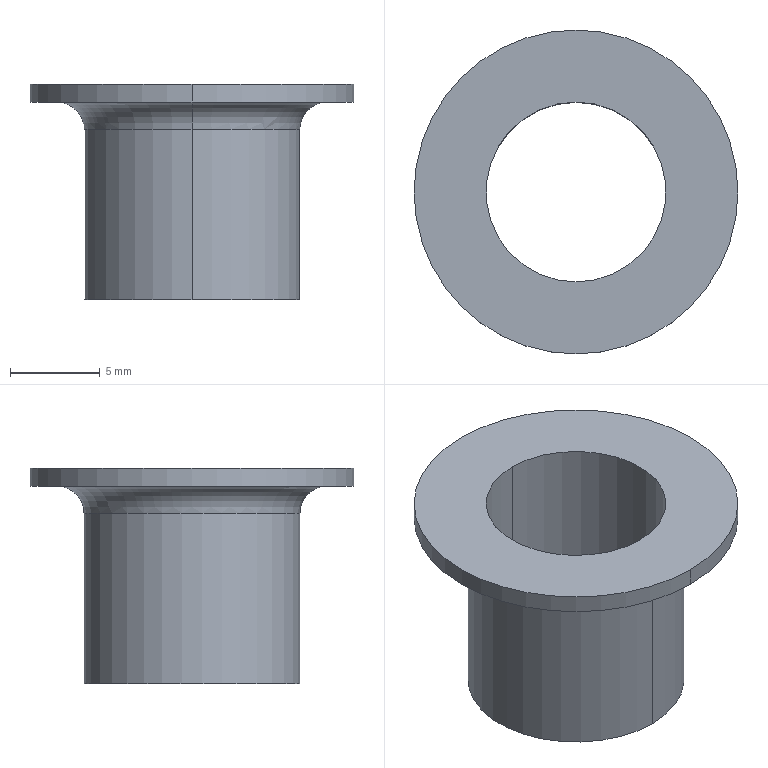Component | SolidWorks | C-SFF10120-1 | 1 solid | 11 faces | box 18 x 18 x 12 mm | volume 575 mm3 | cylinder 6 | plane 3 | torus 2 | commonest cylinder face diameters 12 x2 18 x2 10 x2 | material Tin Bronze
build123d program:
from build123d import *

# Parameters (mm, degrees)
FILLET1_R = 1.5


with BuildPart() as part:
    # Sketch1 → Revolve1 (revolve)
    with BuildSketch(Plane(origin=(0, 0, 0), x_dir=(0, 0, -1), z_dir=(1, 0, 0)), mode=Mode.PRIVATE) as revolve1_sk:
        Polygon((-5, 0), (-9, 0), (-9, 1), (-6, 1), (-6, 12), (-5, 12), align=None)
    revolve(revolve1_sk.sketch.rotate(Axis((0, 0, 0), (0, 1, 0)), 180), axis=Axis((0, 0, 0), (0, 1, 0)))

    # Fillet1
    fillet1_edges = [part.edges().sort_by_distance(p)[0] for p in [
        (0, 1, 6),
    ]]
    fillet(fillet1_edges, radius=FILLET1_R)


solid = part.part

# Placed as in the assembly
solid = solid.moved(Location((31.561, -84.186, 318), (-90, 0, 0)))
STEP:
#1=CARTESIAN_POINT('',(1.243,-3.019,12.48));
#2=VERTEX_POINT('',#1);
#3=CARTESIAN_POINT('',(1.243,-3.61,12.48));
#4=VERTEX_POINT('',#3);
#5=CARTESIAN_POINT('',(1.243,-3.314,12.48));
#6=DIRECTION('',(0.,0.,1.));
#7=DIRECTION('',(0.,-1.,0.));
#8=AXIS2_PLACEMENT_3D('',#5,#6,#7);
#9=CIRCLE('',#8,0.2953);
#10=EDGE_CURVE('',#2,#4,#9,.T.);
#11=ORIENTED_EDGE('',*,*,#10,.F.);
#12=CARTESIAN_POINT('',(1.243,-3.078,12.421));
#13=VERTEX_POINT('',#12);
#14=CARTESIAN_POINT('',(1.243,-3.019,12.421));
#15=DIRECTION('',(1.,-0.,0.));
#16=DIRECTION('',(0.,1.,0.));
#17=AXIS2_PLACEMENT_3D('',#14,#15,#16);
#18=CIRCLE('',#17,0.05906);
#19=EDGE_CURVE('',#2,#13,#18,.T.);
#20=ORIENTED_EDGE('',*,*,#19,.T.);
#21=CARTESIAN_POINT('',(1.243,-3.551,12.421));
#22=VERTEX_POINT('',#21);
#23=CARTESIAN_POINT('',(1.243,-3.314,12.421));
#24=DIRECTION('',(0.,0.,-1.));
#25=DIRECTION('',(0.,-1.,0.));
#26=AXIS2_PLACEMENT_3D('',#23,#24,#25);
#27=CIRCLE('',#26,0.2362);
#28=EDGE_CURVE('',#22,#13,#27,.T.);
#29=ORIENTED_EDGE('',*,*,#28,.F.);
#30=CARTESIAN_POINT('',(1.243,-3.61,12.421));
#31=DIRECTION('',(-1.,0.,0.));
#32=DIRECTION('',(0.,0.,1.));
#33=AXIS2_PLACEMENT_3D('',#30,#31,#32);
#34=CIRCLE('',#33,0.05906);
#35=EDGE_CURVE('',#4,#22,#34,.T.);
#36=ORIENTED_EDGE('',*,*,#35,.F.);
#37=EDGE_LOOP('',(#11,#20,#29,#36));
#38=FACE_OUTER_BOUND('',#37,.T.);
#39=CARTESIAN_POINT('',(1.243,-3.314,12.421));
#40=DIRECTION('',(0.,0.,1.));
#41=DIRECTION('',(0.,-1.,0.));
#42=AXIS2_PLACEMENT_3D('',#39,#40,#41);
#43=TOROIDAL_SURFACE('',#42,0.2953,0.05906);
#44=ADVANCED_FACE('',(#38),#43,.F.);
#45=CARTESIAN_POINT('',(1.243,-3.551,12.047));
#46=VERTEX_POINT('',#45);
#47=CARTESIAN_POINT('',(1.243,-3.078,12.047));
#48=VERTEX_POINT('',#47);
#49=CARTESIAN_POINT('',(1.243,-3.314,12.047));
#50=DIRECTION('',(0.,0.,1.));
#51=DIRECTION('',(0.,-1.,0.));
#52=AXIS2_PLACEMENT_3D('',#49,#50,#51);
#53=CIRCLE('',#52,0.2362);
#54=EDGE_CURVE('',#46,#48,#53,.T.);
#55=ORIENTED_EDGE('',*,*,#54,.T.);
#56=CARTESIAN_POINT('',(1.243,-3.078,12.52));
#57=DIRECTION('',(0.,0.,1.));
#58=VECTOR('',#57,39.37);
#59=LINE('',#56,#58);
#60=EDGE_CURVE('',#48,#13,#59,.T.);
#61=ORIENTED_EDGE('',*,*,#60,.T.);
#62=CARTESIAN_POINT('',(1.243,-3.314,12.421));
#63=DIRECTION('',(0.,0.,-1.));
#64=DIRECTION('',(0.,-1.,0.));
#65=AXIS2_PLACEMENT_3D('',#62,#63,#64);
#66=CIRCLE('',#65,0.2362);
#67=EDGE_CURVE('',#13,#22,#66,.T.);
#68=ORIENTED_EDGE('',*,*,#67,.T.);
#69=CARTESIAN_POINT('',(1.243,-3.551,12.52));
#70=DIRECTION('',(0.,0.,1.));
#71=VECTOR('',#70,39.37);
#72=LINE('',#69,#71);
#73=EDGE_CURVE('',#46,#22,#72,.T.);
#74=ORIENTED_EDGE('',*,*,#73,.F.);
#75=EDGE_LOOP('',(#55,#61,#68,#74));
#76=FACE_OUTER_BOUND('',#75,.T.);
#77=CARTESIAN_POINT('',(1.243,-3.314,12.52));
#78=DIRECTION('',(0.,0.,1.));
#79=DIRECTION('',(0.,-1.,0.));
#80=AXIS2_PLACEMENT_3D('',#77,#78,#79);
#81=CYLINDRICAL_SURFACE('',#80,0.2362);
#82=ADVANCED_FACE('',(#76),#81,.T.);
#83=CARTESIAN_POINT('',(1.243,-3.669,12.48));
#84=VERTEX_POINT('',#83);
#85=CARTESIAN_POINT('',(1.243,-2.96,12.48));
#86=VERTEX_POINT('',#85);
#87=CARTESIAN_POINT('',(1.243,-3.314,12.48));
#88=DIRECTION('',(0.,0.,1.));
#89=DIRECTION('',(0.,-1.,0.));
#90=AXIS2_PLACEMENT_3D('',#87,#88,#89);
#91=CIRCLE('',#90,0.3543);
#92=EDGE_CURVE('',#84,#86,#91,.T.);
#93=ORIENTED_EDGE('',*,*,#92,.T.);
#94=CARTESIAN_POINT('',(1.243,-2.96,12.52));
#95=VERTEX_POINT('',#94);
#96=CARTESIAN_POINT('',(1.243,-2.96,12.52));
#97=DIRECTION('',(0.,0.,1.));
#98=VECTOR('',#97,39.37);
#99=LINE('',#96,#98);
#100=EDGE_CURVE('',#86,#95,#99,.T.);
#101=ORIENTED_EDGE('',*,*,#100,.T.);
#102=CARTESIAN_POINT('',(1.243,-3.669,12.52));
#103=VERTEX_POINT('',#102);
#104=CARTESIAN_POINT('',(1.243,-3.314,12.52));
#105=DIRECTION('',(0.,0.,1.));
#106=DIRECTION('',(0.,-1.,0.));
#107=AXIS2_PLACEMENT_3D('',#104,#105,#106);
#108=CIRCLE('',#107,0.3543);
#109=EDGE_CURVE('',#103,#95,#108,.T.);
#110=ORIENTED_EDGE('',*,*,#109,.F.);
#111=CARTESIAN_POINT('',(1.243,-3.669,12.52));
#112=DIRECTION('',(0.,0.,1.));
#113=VECTOR('',#112,39.37);
#114=LINE('',#111,#113);
#115=EDGE_CURVE('',#84,#103,#114,.T.);
#116=ORIENTED_EDGE('',*,*,#115,.F.);
#117=EDGE_LOOP('',(#93,#101,#110,#116));
#118=FACE_OUTER_BOUND('',#117,.T.);
#119=CARTESIAN_POINT('',(1.243,-3.314,12.52));
#120=DIRECTION('',(0.,0.,1.));
#121=DIRECTION('',(0.,-1.,0.));
#122=AXIS2_PLACEMENT_3D('',#119,#120,#121);
#123=CYLINDRICAL_SURFACE('',#122,0.3543);
#124=ADVANCED_FACE('',(#118),#123,.T.);
#125=CARTESIAN_POINT('',(1.243,-3.118,12.047));
#126=VERTEX_POINT('',#125);
#127=CARTESIAN_POINT('',(1.243,-3.511,12.047));
#128=VERTEX_POINT('',#127);
#129=CARTESIAN_POINT('',(1.243,-3.314,12.047));
#130=DIRECTION('',(0.,0.,1.));
#131=DIRECTION('',(0.,-1.,0.));
#132=AXIS2_PLACEMENT_3D('',#129,#130,#131);
#133=CIRCLE('',#132,0.1969);
#134=EDGE_CURVE('',#126,#128,#133,.T.);
#135=ORIENTED_EDGE('',*,*,#134,.F.);
#136=CARTESIAN_POINT('',(1.243,-3.118,12.52));
#137=VERTEX_POINT('',#136);
#138=CARTESIAN_POINT('',(1.243,-3.118,12.52));
#139=DIRECTION('',(0.,0.,1.));
#140=VECTOR('',#139,39.37);
#141=LINE('',#138,#140);
#142=EDGE_CURVE('',#126,#137,#141,.T.);
#143=ORIENTED_EDGE('',*,*,#142,.T.);
#144=CARTESIAN_POINT('',(1.243,-3.511,12.52));
#145=VERTEX_POINT('',#144);
#146=CARTESIAN_POINT('',(1.243,-3.314,12.52));
#147=DIRECTION('',(0.,0.,1.));
#148=DIRECTION('',(0.,-1.,0.));
#149=AXIS2_PLACEMENT_3D('',#146,#147,#148);
#150=CIRCLE('',#149,0.1969);
#151=EDGE_CURVE('',#137,#145,#150,.T.);
#152=ORIENTED_EDGE('',*,*,#151,.T.);
#153=CARTESIAN_POINT('',(1.243,-3.511,12.52));
#154=DIRECTION('',(0.,0.,1.));
#155=VECTOR('',#154,39.37);
#156=LINE('',#153,#155);
#157=EDGE_CURVE('',#128,#145,#156,.T.);
#158=ORIENTED_EDGE('',*,*,#157,.F.);
#159=EDGE_LOOP('',(#135,#143,#152,#158));
#160=FACE_OUTER_BOUND('',#159,.T.);
#161=CARTESIAN_POINT('',(1.243,-3.314,12.52));
#162=DIRECTION('',(0.,0.,1.));
#163=DIRECTION('',(0.,-1.,0.));
#164=AXIS2_PLACEMENT_3D('',#161,#162,#163);
#165=CYLINDRICAL_SURFACE('',#164,0.1969);
#166=ADVANCED_FACE('',(#160),#165,.F.);
#167=ORIENTED_EDGE('',*,*,#142,.F.);
#168=CARTESIAN_POINT('',(1.243,-3.314,12.047));
#169=DIRECTION('',(0.,0.,1.));
#170=DIRECTION('',(0.,-1.,0.));
#171=AXIS2_PLACEMENT_3D('',#168,#169,#170);
#172=CIRCLE('',#171,0.1969);
#173=EDGE_CURVE('',#128,#126,#172,.T.);
#174=ORIENTED_EDGE('',*,*,#173,.F.);
#175=ORIENTED_EDGE('',*,*,#157,.T.);
#176=CARTESIAN_POINT('',(1.243,-3.314,12.52));
#177=DIRECTION('',(0.,0.,1.));
#178=DIRECTION('',(0.,-1.,0.));
#179=AXIS2_PLACEMENT_3D('',#176,#177,#178);
#180=CIRCLE('',#179,0.1969);
#181=EDGE_CURVE('',#145,#137,#180,.T.);
#182=ORIENTED_EDGE('',*,*,#181,.T.);
#183=EDGE_LOOP('',(#167,#174,#175,#182));
#184=FACE_OUTER_BOUND('',#183,.T.);
#185=CARTESIAN_POINT('',(1.243,-3.314,12.52));
#186=DIRECTION('',(0.,0.,1.));
#187=DIRECTION('',(0.,-1.,0.));
#188=AXIS2_PLACEMENT_3D('',#185,#186,#187);
#189=CYLINDRICAL_SURFACE('',#188,0.1969);
#190=ADVANCED_FACE('',(#184),#189,.F.);
#191=ORIENTED_EDGE('',*,*,#181,.F.);
#192=ORIENTED_EDGE('',*,*,#151,.F.);
#193=EDGE_LOOP('',(#191,#192));
#194=FACE_BOUND('',#193,.T.);
#195=ORIENTED_EDGE('',*,*,#109,.T.);
#196=CARTESIAN_POINT('',(1.243,-3.314,12.52));
#197=DIRECTION('',(0.,0.,1.));
#198=DIRECTION('',(0.,-1.,0.));
#199=AXIS2_PLACEMENT_3D('',#196,#197,#198);
#200=CIRCLE('',#199,0.3543);
#201=EDGE_CURVE('',#95,#103,#200,.T.);
#202=ORIENTED_EDGE('',*,*,#201,.T.);
#203=EDGE_LOOP('',(#195,#202));
#204=FACE_OUTER_BOUND('',#203,.T.);
#205=CARTESIAN_POINT('',(1.243,-3.118,12.52));
#206=DIRECTION('',(0.,0.,-1.));
#207=DIRECTION('',(0.,1.,0.));
#208=AXIS2_PLACEMENT_3D('',#205,#206,#207);
#209=PLANE('',#208);
#210=ADVANCED_FACE('',(#194,#204),#209,.F.);
#211=ORIENTED_EDGE('',*,*,#100,.F.);
#212=CARTESIAN_POINT('',(1.243,-3.314,12.48));
#213=DIRECTION('',(0.,0.,1.));
#214=DIRECTION('',(0.,-1.,0.));
#215=AXIS2_PLACEMENT_3D('',#212,#213,#214);
#216=CIRCLE('',#215,0.3543);
#217=EDGE_CURVE('',#86,#84,#216,.T.);
#218=ORIENTED_EDGE('',*,*,#217,.T.);
#219=ORIENTED_EDGE('',*,*,#115,.T.);
#220=ORIENTED_EDGE('',*,*,#201,.F.);
#221=EDGE_LOOP('',(#211,#218,#219,#220));
#222=FACE_OUTER_BOUND('',#221,.T.);
#223=CARTESIAN_POINT('',(1.243,-3.314,12.52));
#224=DIRECTION('',(0.,0.,1.));
#225=DIRECTION('',(0.,-1.,0.));
#226=AXIS2_PLACEMENT_3D('',#223,#224,#225);
#227=CYLINDRICAL_SURFACE('',#226,0.3543);
#228=ADVANCED_FACE('',(#222),#227,.T.);
#229=CARTESIAN_POINT('',(1.243,-3.314,12.48));
#230=DIRECTION('',(0.,0.,1.));
#231=DIRECTION('',(0.,-1.,0.));
#232=AXIS2_PLACEMENT_3D('',#229,#230,#231);
#233=CIRCLE('',#232,0.2953);
#234=EDGE_CURVE('',#4,#2,#233,.T.);
#235=ORIENTED_EDGE('',*,*,#234,.T.);
#236=ORIENTED_EDGE('',*,*,#10,.T.);
#237=EDGE_LOOP('',(#235,#236));
#238=FACE_BOUND('',#237,.T.);
#239=ORIENTED_EDGE('',*,*,#92,.F.);
#240=ORIENTED_EDGE('',*,*,#217,.F.);
#241=EDGE_LOOP('',(#239,#240));
#242=FACE_OUTER_BOUND('',#241,.T.);
#243=CARTESIAN_POINT('',(1.243,-2.96,12.48));
#244=DIRECTION('',(0.,0.,1.));
#245=DIRECTION('',(0.,-1.,0.));
#246=AXIS2_PLACEMENT_3D('',#243,#244,#245);
#247=PLANE('',#246);
#248=ADVANCED_FACE('',(#238,#242),#247,.F.);
#249=ORIENTED_EDGE('',*,*,#60,.F.);
#250=CARTESIAN_POINT('',(1.243,-3.314,12.047));
#251=DIRECTION('',(0.,0.,1.));
#252=DIRECTION('',(0.,-1.,0.));
#253=AXIS2_PLACEMENT_3D('',#250,#251,#252);
#254=CIRCLE('',#253,0.2362);
#255=EDGE_CURVE('',#48,#46,#254,.T.);
#256=ORIENTED_EDGE('',*,*,#255,.T.);
#257=ORIENTED_EDGE('',*,*,#73,.T.);
#258=ORIENTED_EDGE('',*,*,#28,.T.);
#259=EDGE_LOOP('',(#249,#256,#257,#258));
#260=FACE_OUTER_BOUND('',#259,.T.);
#261=CARTESIAN_POINT('',(1.243,-3.314,12.52));
#262=DIRECTION('',(0.,0.,1.));
#263=DIRECTION('',(0.,-1.,0.));
#264=AXIS2_PLACEMENT_3D('',#261,#262,#263);
#265=CYLINDRICAL_SURFACE('',#264,0.2362);
#266=ADVANCED_FACE('',(#260),#265,.T.);
#267=ORIENTED_EDGE('',*,*,#54,.F.);
#268=ORIENTED_EDGE('',*,*,#255,.F.);
#269=EDGE_LOOP('',(#267,#268));
#270=FACE_OUTER_BOUND('',#269,.T.);
#271=ORIENTED_EDGE('',*,*,#173,.T.);
#272=ORIENTED_EDGE('',*,*,#134,.T.);
#273=EDGE_LOOP('',(#271,#272));
#274=FACE_BOUND('',#273,.T.);
#275=CARTESIAN_POINT('',(1.243,-3.078,12.047));
#276=DIRECTION('',(0.,0.,1.));
#277=DIRECTION('',(0.,-1.,0.));
#278=AXIS2_PLACEMENT_3D('',#275,#276,#277);
#279=PLANE('',#278);
#280=ADVANCED_FACE('',(#270,#274),#279,.F.);
#281=ORIENTED_EDGE('',*,*,#19,.F.);
#282=ORIENTED_EDGE('',*,*,#234,.F.);
#283=ORIENTED_EDGE('',*,*,#35,.T.);
#284=ORIENTED_EDGE('',*,*,#67,.F.);
#285=EDGE_LOOP('',(#281,#282,#283,#284));
#286=FACE_OUTER_BOUND('',#285,.T.);
#287=CARTESIAN_POINT('',(1.243,-3.314,12.421));
#288=DIRECTION('',(0.,0.,1.));
#289=DIRECTION('',(0.,-1.,0.));
#290=AXIS2_PLACEMENT_3D('',#287,#288,#289);
#291=TOROIDAL_SURFACE('',#290,0.2953,0.05906);
#292=ADVANCED_FACE('',(#286),#291,.F.);
#293=CLOSED_SHELL('',(#44,#82,#124,#166,#190,#210,#228,#248,#266,#280,#292));
#294=MANIFOLD_SOLID_BREP('',#293);
#295=CARTESIAN_POINT('',(0.,0.,0.));
#296=DIRECTION('',(0.,0.,1.));
#297=DIRECTION('',(1.,0.,0.));
#298=AXIS2_PLACEMENT_3D('',#295,#296,#297);
#299=(LENGTH_UNIT()NAMED_UNIT(*)SI_UNIT($,.METRE.));
#300=LENGTH_MEASURE_WITH_UNIT(LENGTH_MEASURE(0.0254),#299);
#301=DIMENSIONAL_EXPONENTS(1.,0.,0.,0.,0.,0.,0.);
#302=(CONVERSION_BASED_UNIT('',#300)LENGTH_UNIT()NAMED_UNIT(#301));
#303=UNCERTAINTY_MEASURE_WITH_UNIT(LENGTH_MEASURE(0.00001),#302,'','');
#304=(NAMED_UNIT(*)PLANE_ANGLE_UNIT()SI_UNIT($,.RADIAN.));
#305=(NAMED_UNIT(*)SI_UNIT($,.STERADIAN.)SOLID_ANGLE_UNIT());
#306=(GEOMETRIC_REPRESENTATION_CONTEXT(3)GLOBAL_UNCERTAINTY_ASSIGNED_CONTEXT((#303))GLOBAL_UNIT_ASSIGNED_CONTEXT((#302,#304,#305))REPRESENTATION_CONTEXT('',''));
#307=ADVANCED_BREP_SHAPE_REPRESENTATION('',(#294,#298),#306);
#308=COLOUR_RGB('',0.7922,0.8196,0.9333);
#309=FILL_AREA_STYLE_COLOUR('',#308);
#310=FILL_AREA_STYLE('',(#309));
#311=SURFACE_STYLE_FILL_AREA(#310);
#312=SURFACE_SIDE_STYLE('',(#311));
#313=SURFACE_STYLE_USAGE(.BOTH.,#312);
#314=PRESENTATION_STYLE_ASSIGNMENT((#313));
#315=STYLED_ITEM('',(#314),#294);
#316=PRESENTATION_LAYER_ASSIGNMENT('','',(#315));
#317=(LENGTH_UNIT()NAMED_UNIT(*)SI_UNIT($,.METRE.));
#318=LENGTH_MEASURE_WITH_UNIT(LENGTH_MEASURE(0.0254),#317);
#319=DIMENSIONAL_EXPONENTS(1.,0.,0.,0.,0.,0.,0.);
#320=(CONVERSION_BASED_UNIT('',#318)LENGTH_UNIT()NAMED_UNIT(#319));
#321=UNCERTAINTY_MEASURE_WITH_UNIT(LENGTH_MEASURE(0.00001),#320,'','');
#322=(NAMED_UNIT(*)PLANE_ANGLE_UNIT()SI_UNIT($,.RADIAN.));
#323=(NAMED_UNIT(*)SI_UNIT($,.STERADIAN.)SOLID_ANGLE_UNIT());
#324=(GEOMETRIC_REPRESENTATION_CONTEXT(3)GLOBAL_UNCERTAINTY_ASSIGNED_CONTEXT((#321))GLOBAL_UNIT_ASSIGNED_CONTEXT((#320,#322,#323))REPRESENTATION_CONTEXT('',''));
#325=MECHANICAL_DESIGN_GEOMETRIC_PRESENTATION_REPRESENTATION('',(#315),#324);